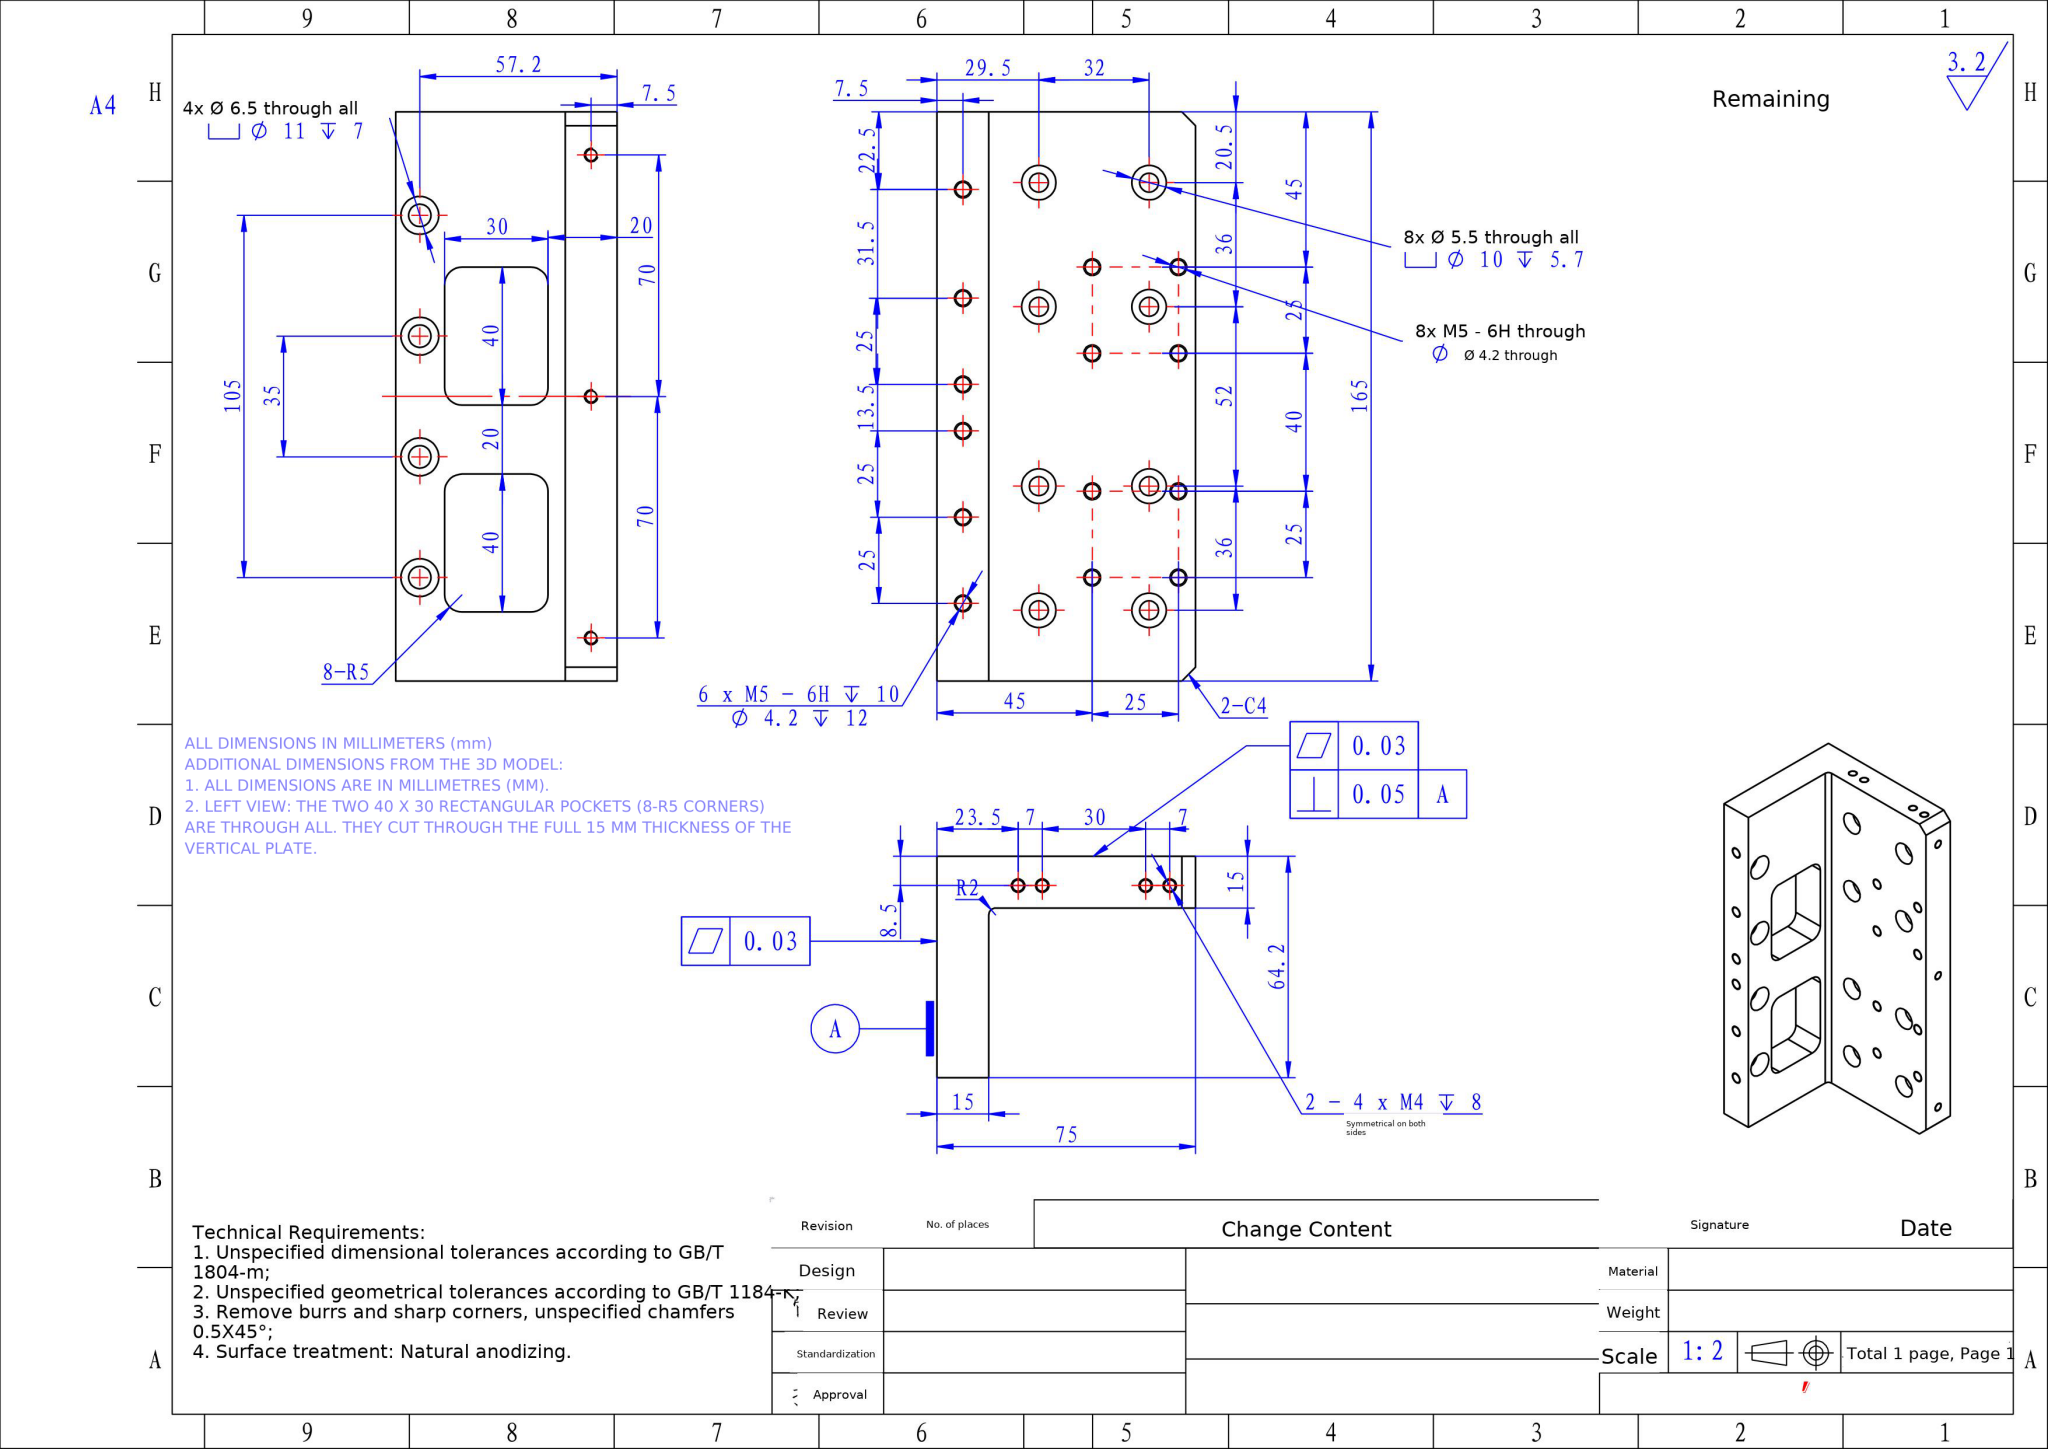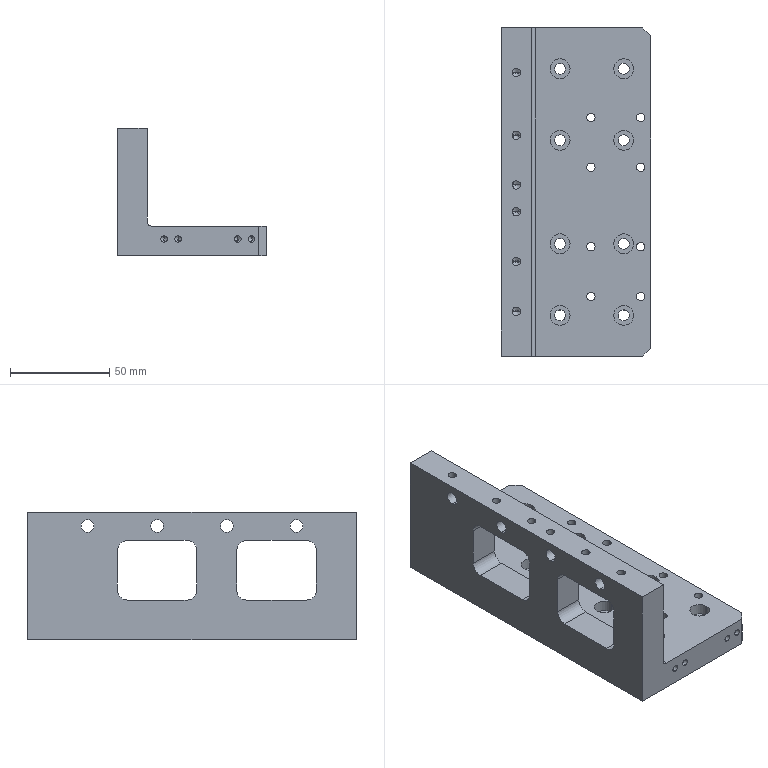Part | NX | mm | Right-Angle Multi-Aperture Perforated Mounting Bracket | 1 solid | 171 faces | box 75 x 165 x 64.2 mm | volume 259181 mm3 | cylinder 107 | cone 34 | plane 30 | commonest cylinder face diameters 4.2 x28 10 x24 3.3 x22 5.5 x16 11 x8 6.5 x8 4 x1